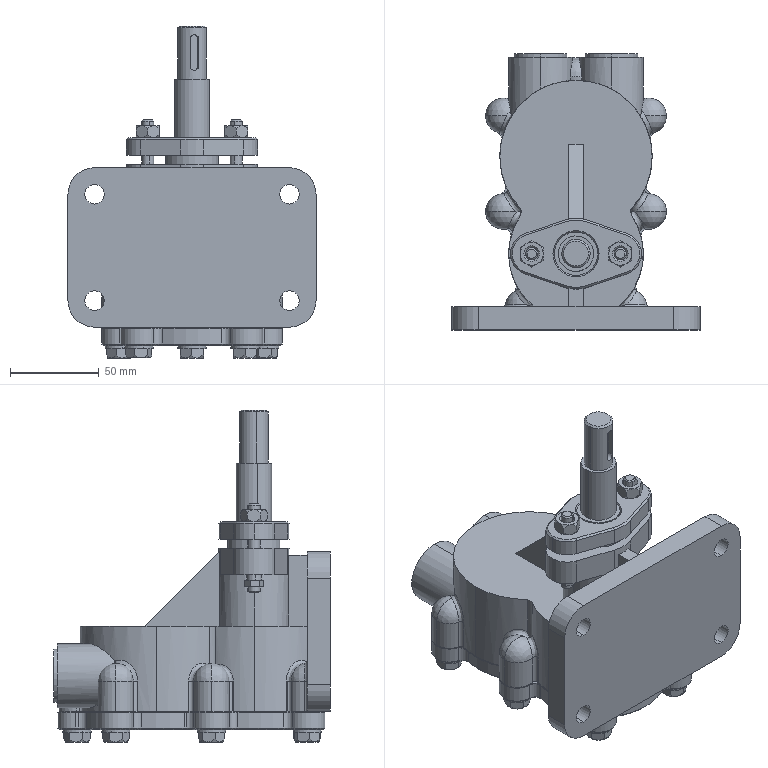Assembly | SolidWorks | mm | 31 component files | 42 solids | 816 faces | box 140 x 156 x 187.4 mm | volume 793396 mm3 | cylinder 370 | plane 212 | cone 198 | torus 16 | sphere 12 | spline 8 | commonest cylinder face diameters 6.8 x70 20 x45 8 x38 10 x28 16 x18 4 x18 25 x16 8.4 x14
Bill of materials:
Bolt | 7 |  | Hex-head bolt-like part: a plain cylindrical shank coming out of a hexagonal head that has chamfered corners.
Bushing | 1 |  | Thin-walled cylindrical sleeve or tube, open at both ends, with one narrow semicircular groove running along the inside wall.
Gasket1 | 1 |  | Very thin flat sheet with a figure-eight outline made of two overlapping circular openings. It has eight lobes around the edge, each with a through-hole.
Gasket2 | 7 |  | Flat annular disc (a washer-like ring) with a central round hole and square, unchamfered edges.
Nut | 2 |  | Hexagonal nut-like body with a central through-bore and chamfered corners on both faces. The bore entry is countersunk or chamfered.
OilSeal | 1 |  | Thin conical ring, like a frustum band: a ring whose outer wall tapers so one face is wider than the other.
Part3 | 1 |  | Short solid cylinder with chamfered end edges and one round cross-hole drilled through it at right angles to the axis.
Part4 | 1 |  | Flanged spigot or boss: a diamond-shaped flange with rounded ends and two small bolt holes, plus a cylindrical boss on one side. A central bore with a chamfered entry runs through both.
Part5Crankshaft | 1 |  | Slender stepped cylindrical shaft/pin. A long main cylindrical body ends in a reduced-diameter end section with what looks like a longitudinal slot or keyway flat. At the other end is a thin integral radial collar (flange), and past it a short smaller-diameter cylindrical stub.
Plunger | 1 |  | Cylindrical pin with chamfered ends, a series of shallow circumferential grooves along part of its length, and a transverse through-hole near one end.
PumpBody | 1 |  | Complex housing-like body. It has a rectangular mounting plate with rounded corners and four corner holes, joined to a body whose outline is two overlapping circles. The body also has a diamond-shaped flanged port with a central bore and two small holes, a cylindrical side boss, rounded lugs around the perimeter, and a sloped gusset.
PumpBodyPartTwo | 1 |  | Thick flat cover plate with a solid figure-eight outline (two overlapping circles) and eight rounded lobes, each with a through-hole. It has small chamfers on the bottom edge.
Stud | 2 |  | Slender solid cylindrical rod/pin with small chamfers at both ends; length roughly 7x its diameter (estimated from the image).
ThinNut | 2 |  | Hexagonal prism with a central circular through-bore; thickness well below the width across flats; flat parallel faces with no visible chamfers.
Washer | 2 |  | Thin-walled cylindrical ring/sleeve with a large concentric through-bore; axial length is about half the outside diameter; plain flat end faces.
Mates:
1. coincident | Gasket2-1 edge at (-39.719, 49.515, 99.5) dir (0, 0, 1) r 8 | assembly plane at (0, 0, 99.5) dir (0, 0, -1)
2. concentric | PumpBodyPartTwo-1 face at (-39.719, 49.515, 99.5) dir (0, 0, 1) r 5 | Gasket2-1 face at (-39.719, 49.515, 99.5) dir (0, 0, -1) r 4.2
3. coincident | Gasket2-1 face at (-39.719, 49.515, 97.9) dir (0, 0, -1) | Bolt-1 face at (-39.719, 49.515, 97.9) dir (0, 0, 1)
4. concentric | PumpBodyPartTwo-1 face at (-39.719, 49.515, 99.5) dir (0, 0, 1) r 5 | Bolt-1 face at (-39.719, 49.515, 122.9) dir (0, 0, -1) r 3.4
5. concentric | PumpBodyPartTwo-1 face at (-80.719, 72.341, 99.5) dir (0, 0, 1) r 5 | Gasket2-2 face at (-80.719, 71.515, 97.9) dir (0, 0, 1) r 8
6. coincident | PumpBodyPartTwo-1 face at (-80.719, 26.515, 99.5) dir (0, 0, -1) | Gasket2-2 face at (-80.719, 71.515, 99.5) dir (0, 0, 1)
7. concentric | PumpBodyPartTwo-1 face at (-121.719, 49.515, 99.5) dir (0, 0, 1) r 5 | Gasket2-3 face at (-121.719, 49.515, 97.9) dir (0, 0, 1) r 8
8. coincident | PumpBodyPartTwo-1 face at (-80.719, 26.515, 109.5) dir (0, 0, 1) | assembly plane at (0, 0, 109.5) dir (0, 0, -1)
9. coincident | Gasket2-2 face at (-80.719, 71.515, 97.9) dir (0, 0, -1) | Bolt-2 face at (-80.719, 71.515, 97.9) dir (0, 0, 1)
10. coincident | Gasket2-3 face at (-121.719, 49.515, 97.9) dir (0, 0, -1) | Bolt-3 face at (-121.719, 49.515, 97.9) dir (0, 0, 1)
11. concentric | PumpBodyPartTwo-1 face at (-39.719, -4.485, 99.5) dir (0, 0, 1) r 5 | Gasket2-5 face at (-39.719, -4.485, 99.5) dir (0, 0, -1) r 4.2
12. coincident | PumpBodyPartTwo-1 face at (-80.719, 26.515, 99.5) dir (0, 0, -1) | Gasket2-5 face at (-39.719, -4.485, 99.5) dir (0, 0, 1)
13. coincident | PumpBodyPartTwo-1 face at (-80.719, 26.515, 99.5) dir (0, 0, -1) | Gasket2-4 face at (-50.719, -58.485, 99.5) dir (0, 0, 1)
14. concentric | PumpBodyPartTwo-1 face at (-50.719, -58.485, 99.5) dir (0, 0, 1) r 5 | Gasket2-4 face at (-50.719, -58.485, 99.5) dir (0, 0, -1) r 4.2
15. concentric | PumpBodyPartTwo-1 face at (-110.719, -58.485, 99.5) dir (0, 0, 1) r 5 | Gasket2-6 face at (-110.719, -58.485, 99.5) dir (0, 0, -1) r 4.2
16. concentric | PumpBodyPartTwo-1 face at (-121.719, -4.485, 99.5) dir (0, 0, 1) r 5 | Gasket2-7 face at (-121.719, -4.485, 99.5) dir (0, 0, -1) r 4.2
17. coincident | Gasket2-5 face at (-39.719, -4.485, 97.9) dir (0, 0, -1) | Bolt-6 face at (-39.719, -4.485, 97.9) dir (0, 0, 1)
18. coincident | PumpBodyPartTwo-1 face at (-80.719, 26.515, 99.5) dir (0, 0, -1) | Gasket2-7 face at (-121.719, -4.485, 99.5) dir (0, 0, 1)
19. coincident | Bolt-5 edge at (-121.719, -4.485, 97.9) dir (0, 0, -1) r 3.8 | Gasket2-7 face at (-121.719, -4.485, 97.9) dir (0, 0, -1)
20. coincident | Bolt-4 face at (-50.719, -58.485, 97.9) dir (0, 0, 1) | Gasket2-4 face at (-50.719, -58.485, 97.9) dir (0, 0, -1)
21. coincident | PumpBodyPartTwo-1 face at (-80.719, 26.515, 99.5) dir (0, 0, -1) | Gasket2-6 face at (-110.719, -58.485, 99.5) dir (0, 0, 1)
22. coincident | Gasket2-6 face at (-110.719, -58.485, 97.9) dir (0, 0, -1) | Bolt-7 face at (-110.719, -58.485, 97.9) dir (0, 0, 1)
23. coincident | Part4-1 face at (-105.719, -28.485, 217) dir (0, 0, 1) | Nut-1 face at (-105.719, -28.485, 217) dir (0, 0, -1)
24. concentric | Nut-1 face at (-105.719, -28.485, 217) dir (0, 0, -1) r 3.4 | Stud-1 face at (-105.719, -28.485, 177.01) dir (0, 0, -1) r 3.4
25. concentric | Bushing-1 face at (-80.719, -28.485, 180) dir (0, 0, -1) r 10 | Part5Crankshaft-1 face at (-80.719, -28.485, 280) dir (0, 0, 1) r 10
26. concentric | Part5Crankshaft-1 face at (-82.499, -18.645, 118) dir (0, 0, 1) r 6.5 | Plunger-1 face at (-82.499, -18.645, 113.5) dir (0, 0, 1) r 6.5
27. concentric | Part3-1 face at (-79.34, 61.488, 130) dir (0.03939, 0.9992, 0) r 12.5 | Plunger-1 face at (-81.101, 16.809, 130) dir (-0.03939, -0.9992, 0) r 12.5
28. concentric | Stud-1 face at (-105.719, -28.485, 177.01) dir (0, 0, -1) r 3.4 | Washer-1 face at (-105.719, -28.485, 184) dir (0, 0, 1) r 4.118
29. distance | Stud-1 face at (-105.719, -28.485, 227.01) dir (0, 0, 1) | Nut-1 face at (-105.719, -28.485, 223.8) dir (0, 0, 1)
30. concentric | Washer-1 face at (-105.719, -28.485, 184) dir (0, 0, 1) r 4.118 | ThinNut-1 face at (-105.719, -28.485, 180.5) dir (0, 0, 1) r 3.4
31. coincident | Washer-1 face at (-105.719, -28.485, 184) dir (0, 0, -1) | ThinNut-1 edge at (-110.119, -31.587, 184) dir (-0.09039, 0.9959, 0)
32. concentric | Part5Crankshaft-1 face at (-80.719, -28.485, 280) dir (0, 0, 1) r 10 | OilSeal-1 face at (-80.719, -28.485, 201.536) dir (0, 0, 1) r 10
33. coincident | Part4-1 edge at (-80.719, -28.485, 213.536) dir (0, 0, 1) r 11 | OilSeal-1 edge at (-80.719, -28.485, 213.536) dir (0, 0, 1) r 11
34. concentric | Bushing-1 face at (-80.719, -28.485, 180) dir (0, 0, -1) r 12.5 | PumpBody-1 face at (-80.719, -28.485, 187) dir (0, 0, 1) r 15
35. concentric | Bolt-3 face at (-121.719, 49.515, 122.9) dir (0, 0, -1) r 3.4 | PumpBody-1 face at (-121.719, 49.515, 110) dir (0, 0, -1) r 3.4
36. coincident | Gasket1-1 face at (-80.719, 26.515, 110) dir (0, 0, 1) | PumpBody-1 face at (-121.719, -4.485, 110) dir (0, 0, -1)